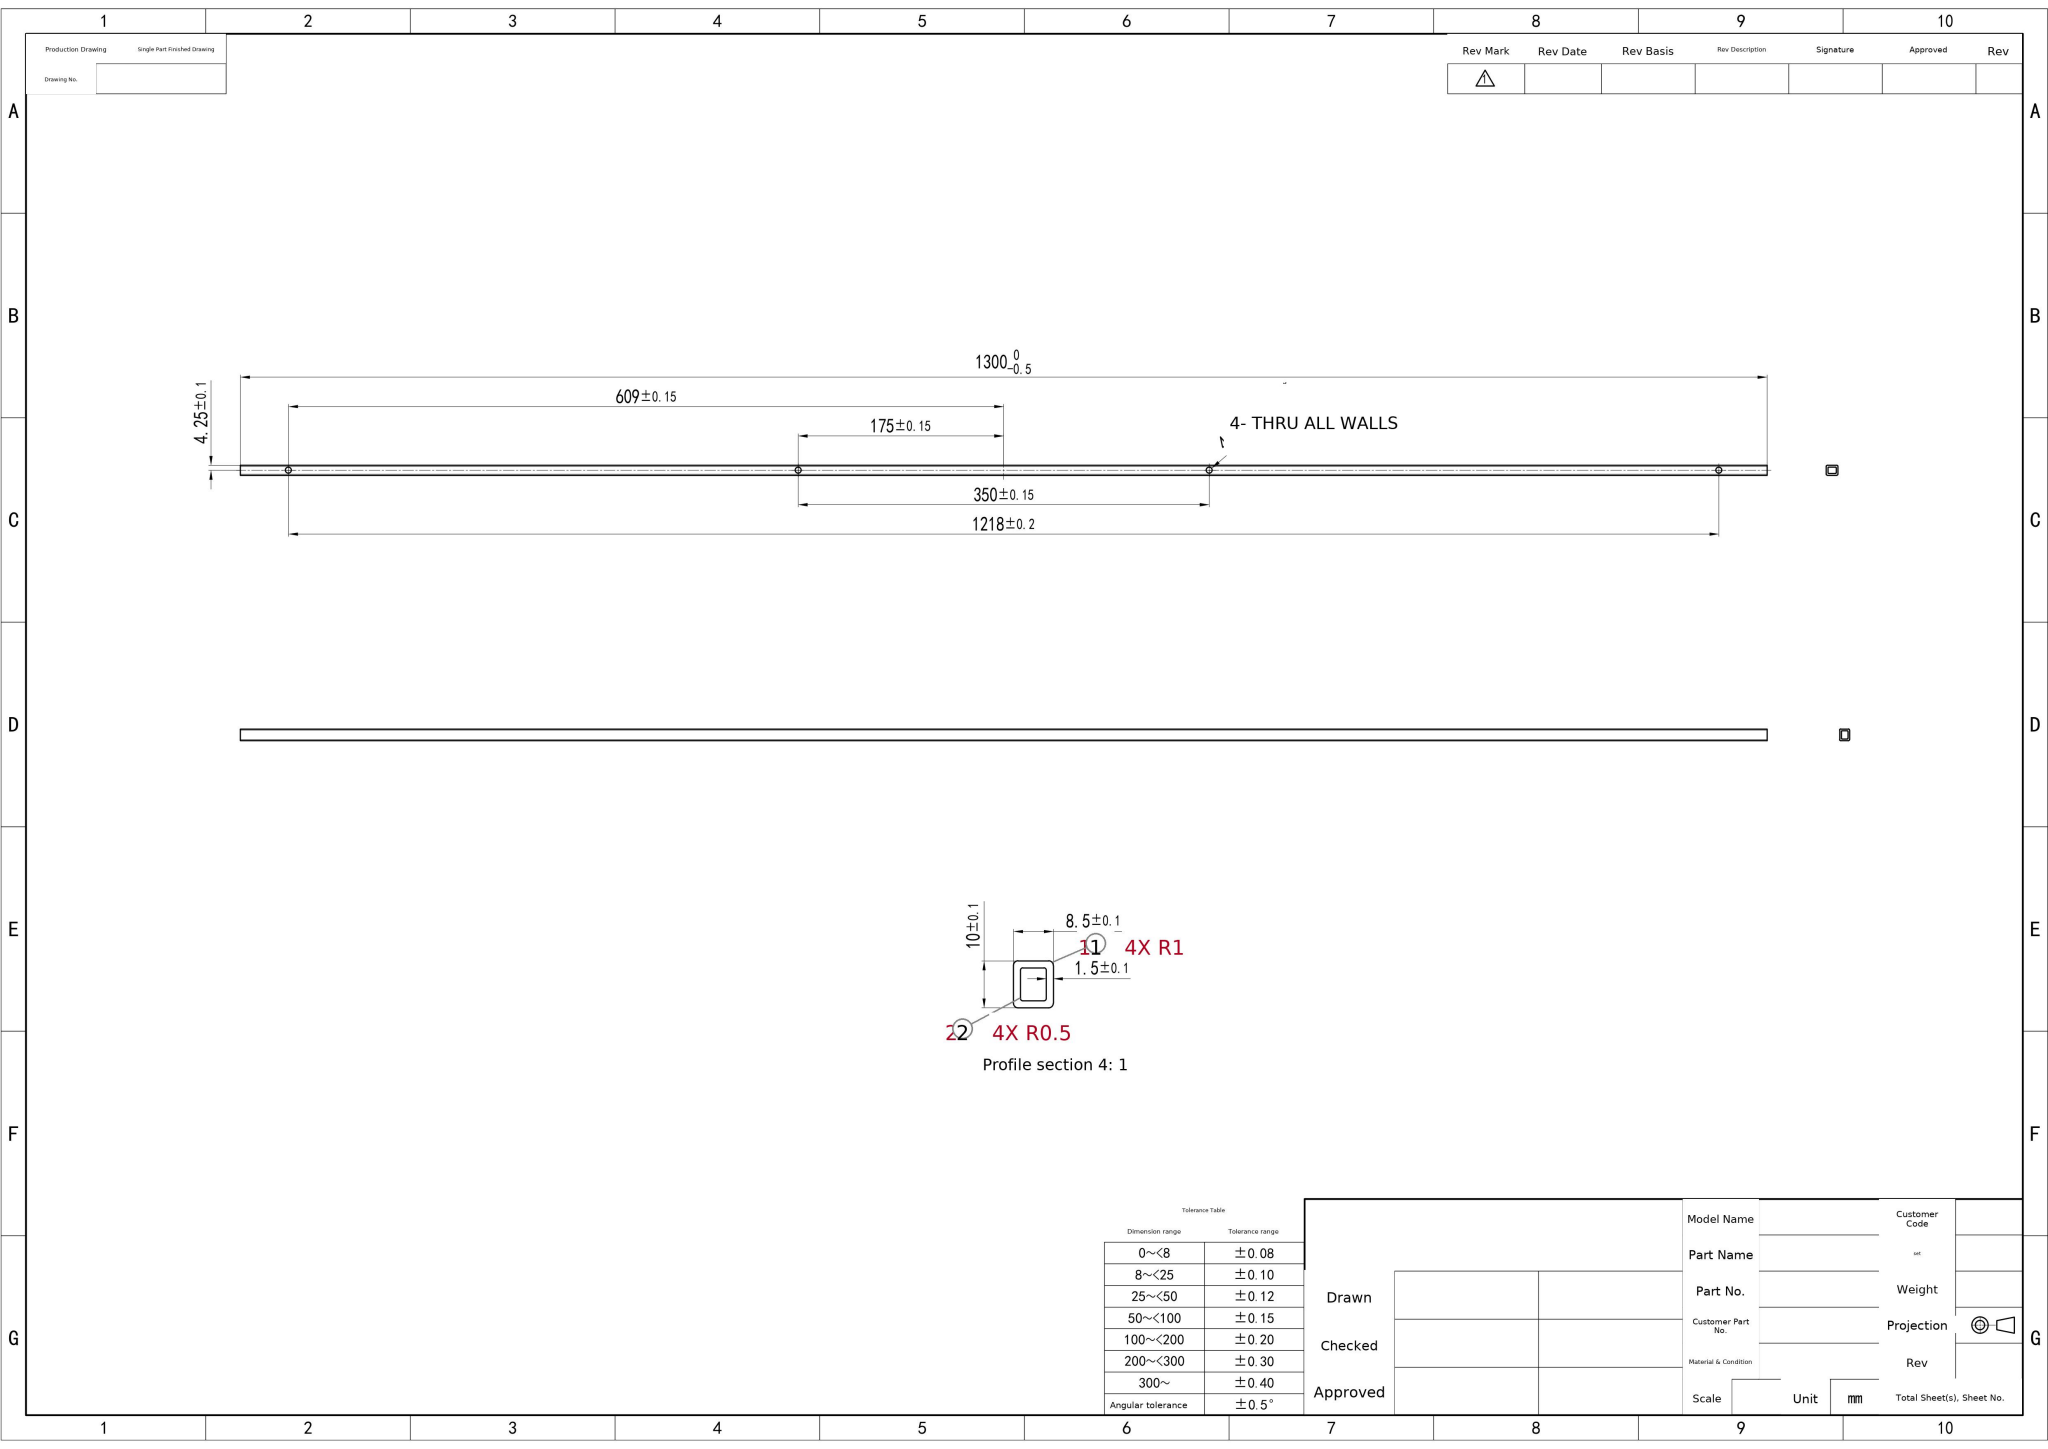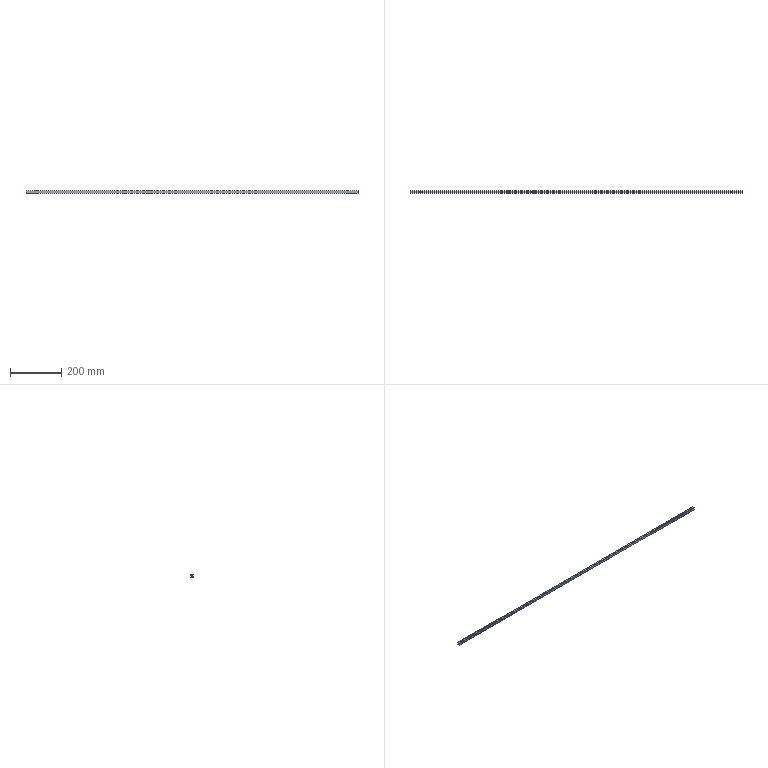Part | SolidWorks | mm | 1 solid | 42 faces | box 1300 x 8.5 x 10 mm | volume 59377 mm3 | cylinder 24 | plane 18 | commonest cylinder face diameters 5 x16 2 x4 1 x4